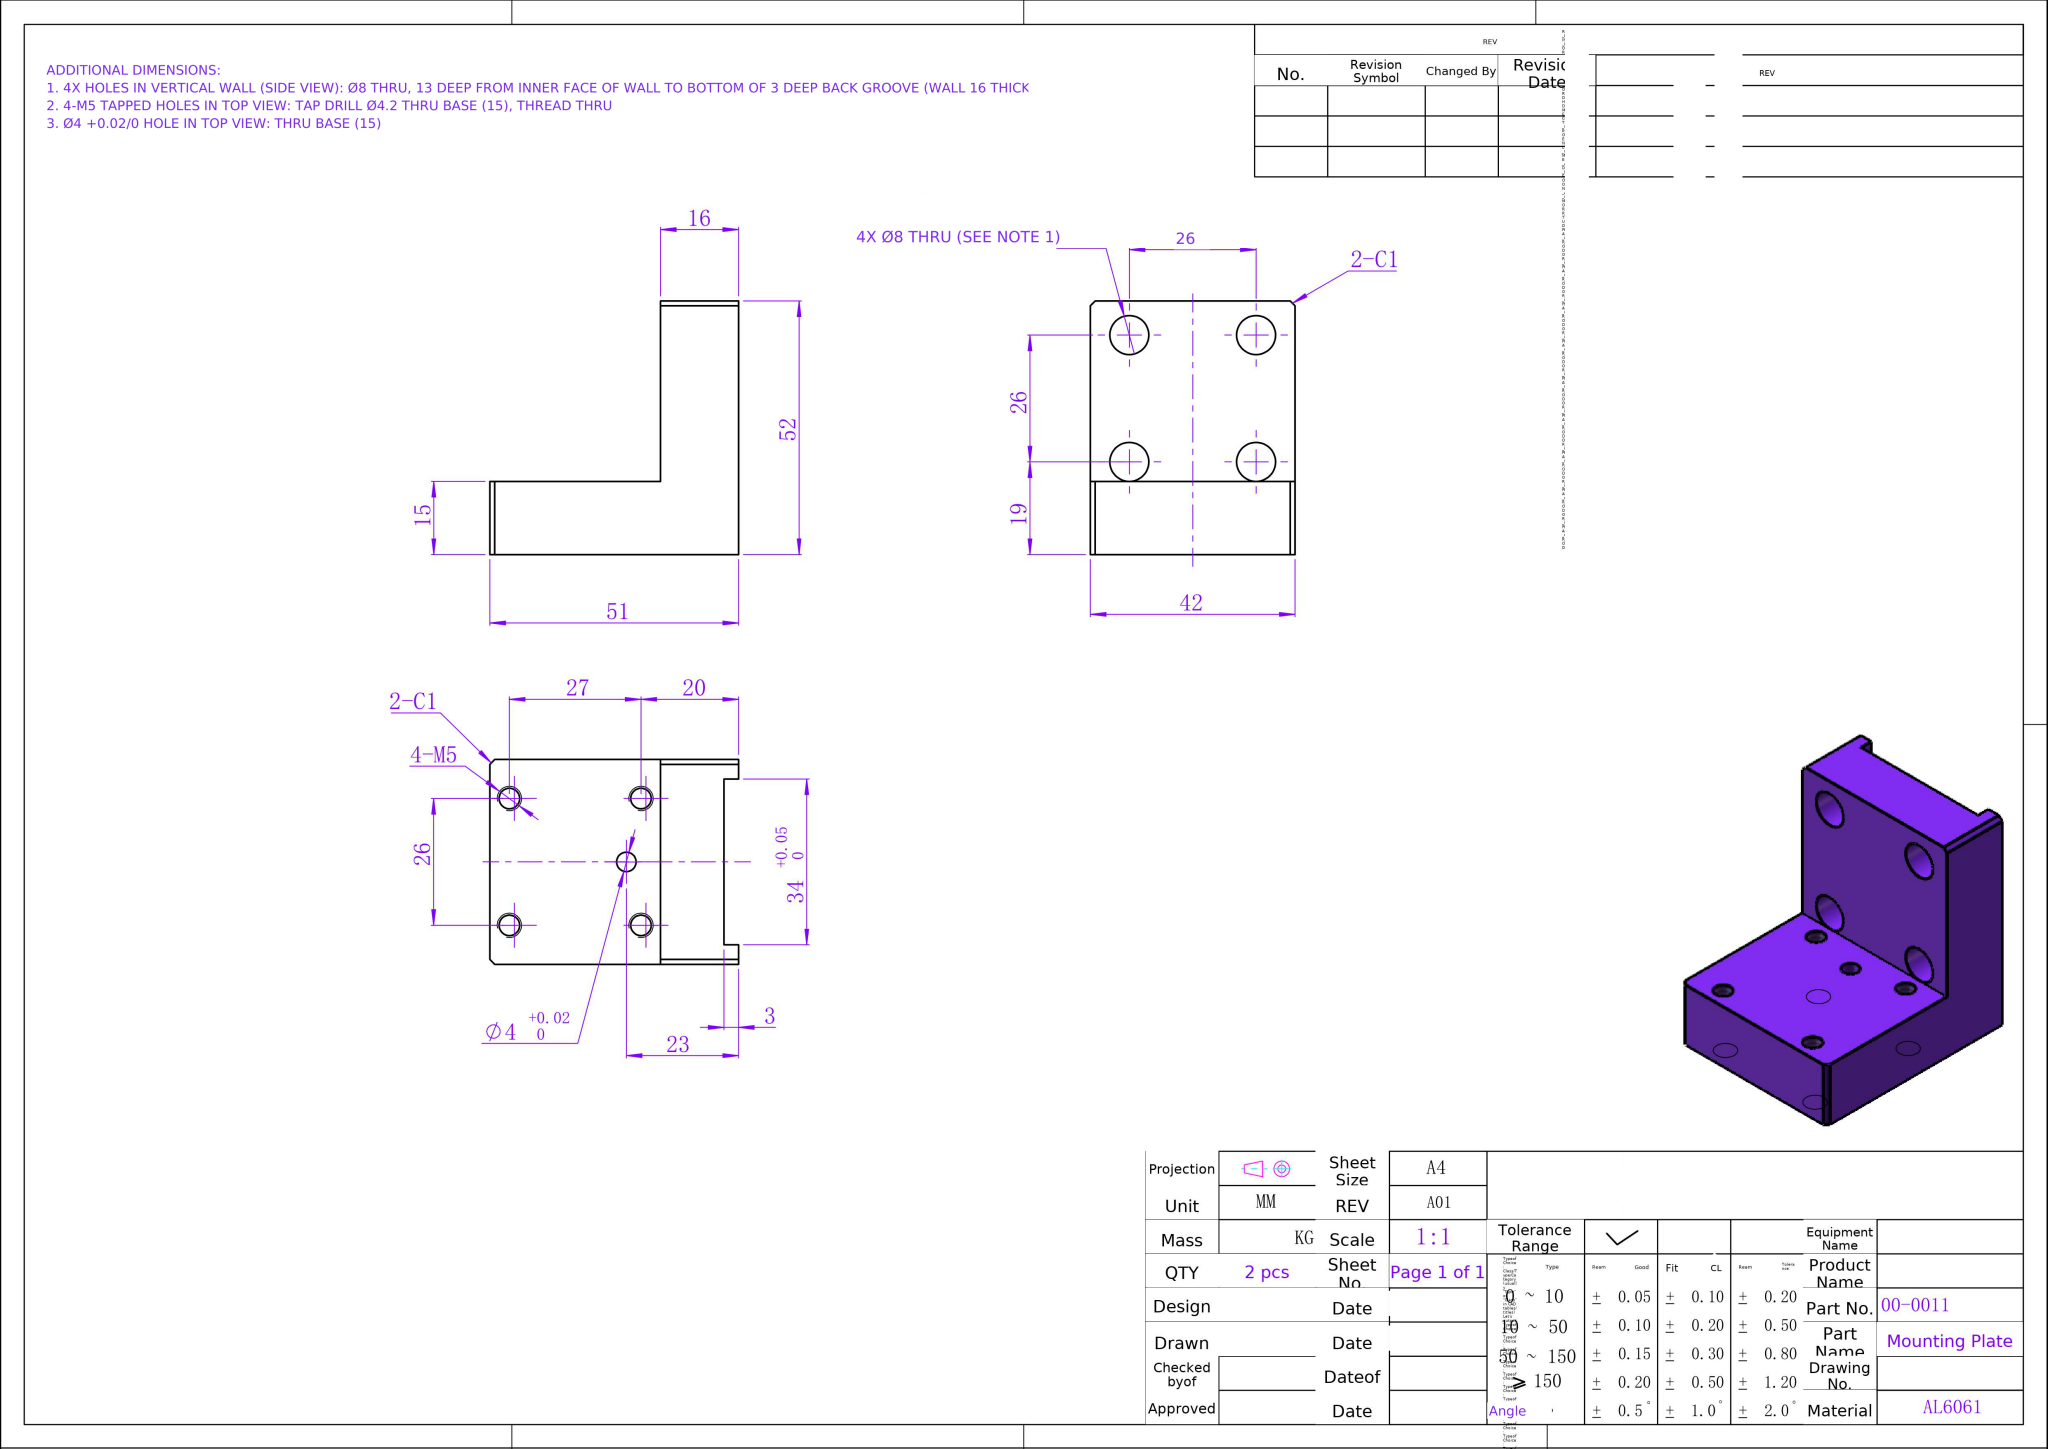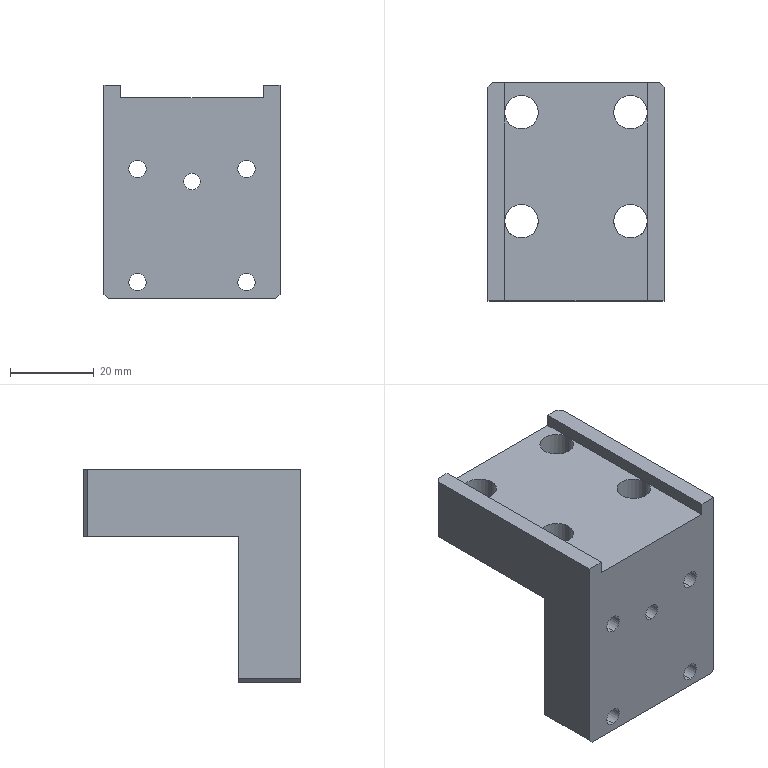Part | NX | mm | 1 solid | 34 faces | box 42 x 52 x 51 mm | volume 48025 mm3 | cylinder 18 | plane 16 | commonest cylinder face diameters 4.2 x8 8 x8 4 x2